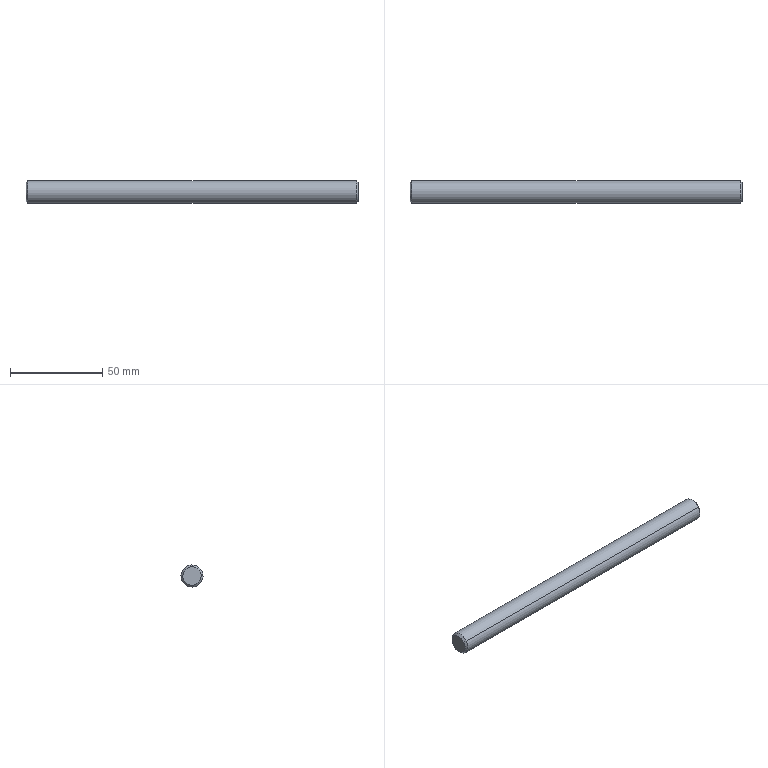Component | SolidWorks | XM-WST05-2006-1 | 1 solid | 8 faces | box 180 x 12 x 12 mm | volume 20322 mm3 | cone 4 | cylinder 2 | plane 2 | commonest cylinder face diameters 12 x2
build123d program:
from build123d import *

# Parameters (mm, degrees)
SKETCH1_R           = 6
BOSS_EXTRUDE1_DEPTH = 180
CHAMFER1_SIZE       = 1


with BuildPart() as part:
    # Sketch1 → Boss-Extrude1 (new body)
    with BuildSketch(Plane.XY):
        with Locations(Location((0, 0, 0), (0, 0, 180))):
            Circle(SKETCH1_R)
    extrude(amount=BOSS_EXTRUDE1_DEPTH)

    # Chamfer1
    chamfer1_edges = [part.edges().sort_by_distance(p)[0] for p in [
        (6, 0, 0),
        (6, 0, 180),
    ]]
    chamfer(chamfer1_edges, length=CHAMFER1_SIZE)


solid = part.part

# Placed as in the assembly
solid = solid.moved(Location((-235.071, 84.169, 359.808), (0, 90, 0)))
STEP:
#1=COLOUR_RGB('',0.7922,0.8196,0.9333);
#2=FILL_AREA_STYLE_COLOUR('',#1);
#3=FILL_AREA_STYLE('',(#2));
#4=SURFACE_STYLE_FILL_AREA(#3);
#5=SURFACE_SIDE_STYLE('',(#4));
#6=SURFACE_STYLE_USAGE(.BOTH.,#5);
#7=PRESENTATION_STYLE_ASSIGNMENT((#6));
#8=CARTESIAN_POINT('',(-2.168,3.158,14.286));
#9=VERTEX_POINT('',#8);
#10=CARTESIAN_POINT('',(-2.168,3.47,14.045));
#11=VERTEX_POINT('',#10);
#12=CARTESIAN_POINT('',(-2.168,3.314,14.166));
#13=DIRECTION('',(1.,0.,-0.));
#14=DIRECTION('',(0.,0.7916,-0.611));
#15=AXIS2_PLACEMENT_3D('',#12,#13,#14);
#16=CIRCLE('',#15,0.1969);
#17=EDGE_CURVE('',#9,#11,#16,.T.);
#18=ORIENTED_EDGE('',*,*,#17,.F.);
#19=CARTESIAN_POINT('',(-2.208,3.127,14.31));
#20=VERTEX_POINT('',#19);
#21=CARTESIAN_POINT('',(-2.208,3.127,14.31));
#22=DIRECTION('',(-0.7071,-0.5598,0.432));
#23=VECTOR('',#22,39.37);
#24=LINE('',#21,#23);
#25=EDGE_CURVE('',#9,#20,#24,.T.);
#26=ORIENTED_EDGE('',*,*,#25,.T.);
#27=CARTESIAN_POINT('',(-2.208,3.501,14.021));
#28=VERTEX_POINT('',#27);
#29=CARTESIAN_POINT('',(-2.208,3.314,14.166));
#30=DIRECTION('',(-1.,-0.,0.));
#31=DIRECTION('',(0.,0.7916,-0.611));
#32=AXIS2_PLACEMENT_3D('',#29,#30,#31);
#33=CIRCLE('',#32,0.2362);
#34=EDGE_CURVE('',#28,#20,#33,.T.);
#35=ORIENTED_EDGE('',*,*,#34,.F.);
#36=CARTESIAN_POINT('',(-2.208,3.501,14.021));
#37=DIRECTION('',(-0.7071,0.5598,-0.432));
#38=VECTOR('',#37,39.37);
#39=LINE('',#36,#38);
#40=EDGE_CURVE('',#11,#28,#39,.T.);
#41=ORIENTED_EDGE('',*,*,#40,.F.);
#42=EDGE_LOOP('',(#18,#26,#35,#41));
#43=FACE_OUTER_BOUND('',#42,.T.);
#44=CARTESIAN_POINT('',(-2.208,3.314,14.166));
#45=DIRECTION('',(-1.,-0.,0.));
#46=DIRECTION('',(0.,0.7916,-0.611));
#47=AXIS2_PLACEMENT_3D('',#44,#45,#46);
#48=CONICAL_SURFACE('',#47,0.2362,0.7854);
#49=ADVANCED_FACE('',(#43),#48,.T.);
#50=CARTESIAN_POINT('',(-9.255,3.47,14.045));
#51=VERTEX_POINT('',#50);
#52=CARTESIAN_POINT('',(-9.255,3.158,14.286));
#53=VERTEX_POINT('',#52);
#54=CARTESIAN_POINT('',(-9.255,3.314,14.166));
#55=DIRECTION('',(-1.,-0.,0.));
#56=DIRECTION('',(0.,0.7916,-0.611));
#57=AXIS2_PLACEMENT_3D('',#54,#55,#56);
#58=CIRCLE('',#57,0.1969);
#59=EDGE_CURVE('',#51,#53,#58,.T.);
#60=ORIENTED_EDGE('',*,*,#59,.F.);
#61=CARTESIAN_POINT('',(-9.215,3.501,14.021));
#62=VERTEX_POINT('',#61);
#63=CARTESIAN_POINT('',(-9.255,3.47,14.045));
#64=DIRECTION('',(0.7071,0.5598,-0.432));
#65=VECTOR('',#64,39.37);
#66=LINE('',#63,#65);
#67=EDGE_CURVE('',#51,#62,#66,.T.);
#68=ORIENTED_EDGE('',*,*,#67,.T.);
#69=CARTESIAN_POINT('',(-9.215,3.127,14.31));
#70=VERTEX_POINT('',#69);
#71=CARTESIAN_POINT('',(-9.215,3.314,14.166));
#72=DIRECTION('',(1.,0.,-0.));
#73=DIRECTION('',(0.,0.7916,-0.611));
#74=AXIS2_PLACEMENT_3D('',#71,#72,#73);
#75=CIRCLE('',#74,0.2362);
#76=EDGE_CURVE('',#70,#62,#75,.T.);
#77=ORIENTED_EDGE('',*,*,#76,.F.);
#78=CARTESIAN_POINT('',(-9.255,3.158,14.286));
#79=DIRECTION('',(0.7071,-0.5598,0.432));
#80=VECTOR('',#79,39.37);
#81=LINE('',#78,#80);
#82=EDGE_CURVE('',#53,#70,#81,.T.);
#83=ORIENTED_EDGE('',*,*,#82,.F.);
#84=EDGE_LOOP('',(#60,#68,#77,#83));
#85=FACE_OUTER_BOUND('',#84,.T.);
#86=CARTESIAN_POINT('',(-9.255,3.314,14.166));
#87=DIRECTION('',(1.,0.,-0.));
#88=DIRECTION('',(0.,-0.7916,0.611));
#89=AXIS2_PLACEMENT_3D('',#86,#87,#88);
#90=CONICAL_SURFACE('',#89,0.1969,0.7854);
#91=ADVANCED_FACE('',(#85),#90,.T.);
#92=ORIENTED_EDGE('',*,*,#76,.T.);
#93=CARTESIAN_POINT('',(-9.255,3.501,14.021));
#94=DIRECTION('',(1.,0.,-0.));
#95=VECTOR('',#94,39.37);
#96=LINE('',#93,#95);
#97=EDGE_CURVE('',#62,#28,#96,.T.);
#98=ORIENTED_EDGE('',*,*,#97,.T.);
#99=ORIENTED_EDGE('',*,*,#34,.T.);
#100=CARTESIAN_POINT('',(-9.255,3.127,14.31));
#101=DIRECTION('',(1.,0.,-0.));
#102=VECTOR('',#101,39.37);
#103=LINE('',#100,#102);
#104=EDGE_CURVE('',#70,#20,#103,.T.);
#105=ORIENTED_EDGE('',*,*,#104,.F.);
#106=EDGE_LOOP('',(#92,#98,#99,#105));
#107=FACE_OUTER_BOUND('',#106,.T.);
#108=CARTESIAN_POINT('',(-9.255,3.314,14.166));
#109=DIRECTION('',(1.,0.,-0.));
#110=DIRECTION('',(0.,-0.7916,0.611));
#111=AXIS2_PLACEMENT_3D('',#108,#109,#110);
#112=CYLINDRICAL_SURFACE('',#111,0.2362);
#113=ADVANCED_FACE('',(#107),#112,.T.);
#114=ORIENTED_EDGE('',*,*,#97,.F.);
#115=CARTESIAN_POINT('',(-9.215,3.314,14.166));
#116=DIRECTION('',(1.,0.,-0.));
#117=DIRECTION('',(0.,0.7916,-0.611));
#118=AXIS2_PLACEMENT_3D('',#115,#116,#117);
#119=CIRCLE('',#118,0.2362);
#120=EDGE_CURVE('',#62,#70,#119,.T.);
#121=ORIENTED_EDGE('',*,*,#120,.T.);
#122=ORIENTED_EDGE('',*,*,#104,.T.);
#123=CARTESIAN_POINT('',(-2.208,3.314,14.166));
#124=DIRECTION('',(-1.,-0.,0.));
#125=DIRECTION('',(0.,0.7916,-0.611));
#126=AXIS2_PLACEMENT_3D('',#123,#124,#125);
#127=CIRCLE('',#126,0.2362);
#128=EDGE_CURVE('',#20,#28,#127,.T.);
#129=ORIENTED_EDGE('',*,*,#128,.T.);
#130=EDGE_LOOP('',(#114,#121,#122,#129));
#131=FACE_OUTER_BOUND('',#130,.T.);
#132=CARTESIAN_POINT('',(-9.255,3.314,14.166));
#133=DIRECTION('',(1.,0.,-0.));
#134=DIRECTION('',(0.,-0.7916,0.611));
#135=AXIS2_PLACEMENT_3D('',#132,#133,#134);
#136=CYLINDRICAL_SURFACE('',#135,0.2362);
#137=ADVANCED_FACE('',(#131),#136,.T.);
#138=CARTESIAN_POINT('',(-9.255,3.314,14.166));
#139=DIRECTION('',(-1.,-0.,0.));
#140=DIRECTION('',(0.,0.7916,-0.611));
#141=AXIS2_PLACEMENT_3D('',#138,#139,#140);
#142=CIRCLE('',#141,0.1969);
#143=EDGE_CURVE('',#53,#51,#142,.T.);
#144=ORIENTED_EDGE('',*,*,#143,.T.);
#145=ORIENTED_EDGE('',*,*,#59,.T.);
#146=EDGE_LOOP('',(#144,#145));
#147=FACE_OUTER_BOUND('',#146,.T.);
#148=CARTESIAN_POINT('',(-9.255,3.314,14.166));
#149=DIRECTION('',(-1.,-0.,0.));
#150=DIRECTION('',(-0.,0.7916,-0.611));
#151=AXIS2_PLACEMENT_3D('',#148,#149,#150);
#152=PLANE('',#151);
#153=ADVANCED_FACE('',(#147),#152,.T.);
#154=CARTESIAN_POINT('',(-2.168,3.314,14.166));
#155=DIRECTION('',(1.,0.,-0.));
#156=DIRECTION('',(0.,0.7916,-0.611));
#157=AXIS2_PLACEMENT_3D('',#154,#155,#156);
#158=CIRCLE('',#157,0.1969);
#159=EDGE_CURVE('',#11,#9,#158,.T.);
#160=ORIENTED_EDGE('',*,*,#159,.T.);
#161=ORIENTED_EDGE('',*,*,#17,.T.);
#162=EDGE_LOOP('',(#160,#161));
#163=FACE_OUTER_BOUND('',#162,.T.);
#164=CARTESIAN_POINT('',(-2.168,3.314,14.166));
#165=DIRECTION('',(-1.,-0.,0.));
#166=DIRECTION('',(-0.,0.7916,-0.611));
#167=AXIS2_PLACEMENT_3D('',#164,#165,#166);
#168=PLANE('',#167);
#169=ADVANCED_FACE('',(#163),#168,.F.);
#170=ORIENTED_EDGE('',*,*,#67,.F.);
#171=ORIENTED_EDGE('',*,*,#143,.F.);
#172=ORIENTED_EDGE('',*,*,#82,.T.);
#173=ORIENTED_EDGE('',*,*,#120,.F.);
#174=EDGE_LOOP('',(#170,#171,#172,#173));
#175=FACE_OUTER_BOUND('',#174,.T.);
#176=CARTESIAN_POINT('',(-9.255,3.314,14.166));
#177=DIRECTION('',(1.,0.,-0.));
#178=DIRECTION('',(0.,-0.7916,0.611));
#179=AXIS2_PLACEMENT_3D('',#176,#177,#178);
#180=CONICAL_SURFACE('',#179,0.1969,0.7854);
#181=ADVANCED_FACE('',(#175),#180,.T.);
#182=ORIENTED_EDGE('',*,*,#25,.F.);
#183=ORIENTED_EDGE('',*,*,#159,.F.);
#184=ORIENTED_EDGE('',*,*,#40,.T.);
#185=ORIENTED_EDGE('',*,*,#128,.F.);
#186=EDGE_LOOP('',(#182,#183,#184,#185));
#187=FACE_OUTER_BOUND('',#186,.T.);
#188=CARTESIAN_POINT('',(-2.208,3.314,14.166));
#189=DIRECTION('',(-1.,-0.,0.));
#190=DIRECTION('',(0.,0.7916,-0.611));
#191=AXIS2_PLACEMENT_3D('',#188,#189,#190);
#192=CONICAL_SURFACE('',#191,0.2362,0.7854);
#193=ADVANCED_FACE('',(#187),#192,.T.);
#194=CLOSED_SHELL('',(#49,#91,#113,#137,#153,#169,#181,#193));
#195=MANIFOLD_SOLID_BREP('',#194);
#196=STYLED_ITEM('',(#7),#195);
#197=(LENGTH_UNIT()NAMED_UNIT(*)SI_UNIT($,.METRE.));
#198=LENGTH_MEASURE_WITH_UNIT(LENGTH_MEASURE(0.0254),#197);
#199=DIMENSIONAL_EXPONENTS(1.,0.,0.,0.,0.,0.,0.);
#200=(CONVERSION_BASED_UNIT('',#198)LENGTH_UNIT()NAMED_UNIT(#199));
#201=UNCERTAINTY_MEASURE_WITH_UNIT(LENGTH_MEASURE(0.00001),#200,'','');
#202=(NAMED_UNIT(*)PLANE_ANGLE_UNIT()SI_UNIT($,.RADIAN.));
#203=(NAMED_UNIT(*)SI_UNIT($,.STERADIAN.)SOLID_ANGLE_UNIT());
#204=(GEOMETRIC_REPRESENTATION_CONTEXT(3)GLOBAL_UNCERTAINTY_ASSIGNED_CONTEXT((#201))GLOBAL_UNIT_ASSIGNED_CONTEXT((#200,#202,#203))REPRESENTATION_CONTEXT('',''));
#205=MECHANICAL_DESIGN_GEOMETRIC_PRESENTATION_REPRESENTATION('',(#196),#204);
#206=CARTESIAN_POINT('',(0.,0.,0.));
#207=DIRECTION('',(0.,0.,1.));
#208=DIRECTION('',(1.,0.,0.));
#209=AXIS2_PLACEMENT_3D('',#206,#207,#208);
#210=(LENGTH_UNIT()NAMED_UNIT(*)SI_UNIT($,.METRE.));
#211=LENGTH_MEASURE_WITH_UNIT(LENGTH_MEASURE(0.0254),#210);
#212=DIMENSIONAL_EXPONENTS(1.,0.,0.,0.,0.,0.,0.);
#213=(CONVERSION_BASED_UNIT('',#211)LENGTH_UNIT()NAMED_UNIT(#212));
#214=UNCERTAINTY_MEASURE_WITH_UNIT(LENGTH_MEASURE(0.00001),#213,'','');
#215=(NAMED_UNIT(*)PLANE_ANGLE_UNIT()SI_UNIT($,.RADIAN.));
#216=(NAMED_UNIT(*)SI_UNIT($,.STERADIAN.)SOLID_ANGLE_UNIT());
#217=(GEOMETRIC_REPRESENTATION_CONTEXT(3)GLOBAL_UNCERTAINTY_ASSIGNED_CONTEXT((#214))GLOBAL_UNIT_ASSIGNED_CONTEXT((#213,#215,#216))REPRESENTATION_CONTEXT('',''));
#218=ADVANCED_BREP_SHAPE_REPRESENTATION('',(#195,#209),#217);
#219=PRESENTATION_LAYER_ASSIGNMENT('','',(#196));